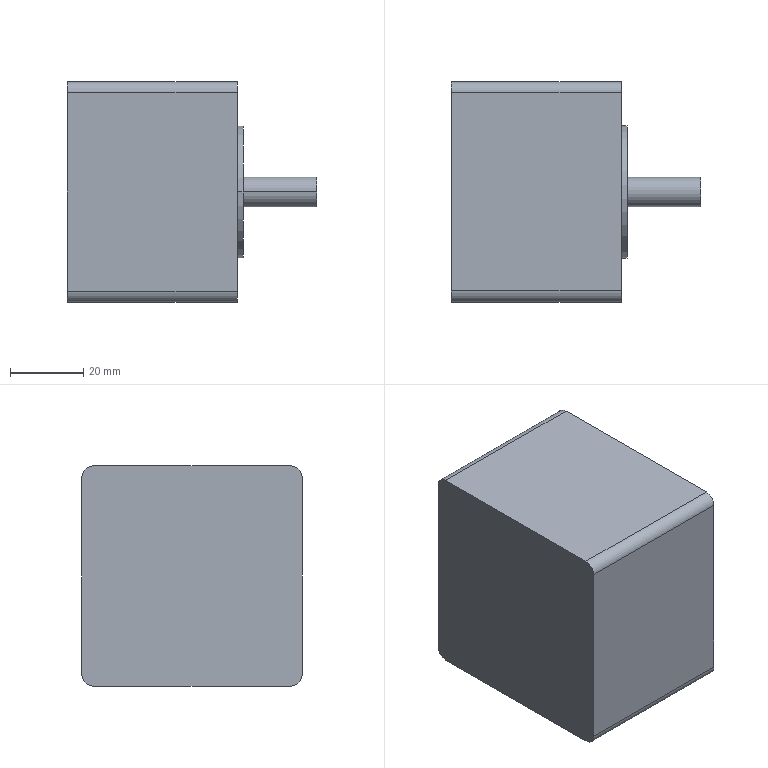Component | SolidWorks | 60Step-1 | 1 solid | 32 faces | box 67.9 x 60 x 60 mm | volume 168599 mm3 | cylinder 16 | cone 8 | plane 8 | commonest cylinder face diameters 3.3 x8 6 x4 8 x2 36 x2
build123d program:
from build123d import *

# Parameters (mm, degrees)
SKETCH1_W             = 60
SKETCH1_H             = 60
BOSS_EXTRUDE1_DEPTH   = 46.3
SKETCH2_R             = 18
BOSS_EXTRUDE2_DEPTH   = 1.6
M4_TAPPED_HOLE1_D     = 3.3
M4_TAPPED_HOLE1_DEPTH = 10.1
M4_TAPPED_HOLE1_TIP   = 0.9914
SKETCH6_R             = 4
BOSS_EXTRUDE3_DEPTH   = 20
FILLET1_R             = 3


with BuildPart() as part:
    # Sketch1 → Boss-Extrude1 (new body)
    with BuildSketch(Plane.XY):
        Rectangle(SKETCH1_W, SKETCH1_H)
    extrude(amount=BOSS_EXTRUDE1_DEPTH)

    # Sketch2 → Boss-Extrude2 (add)
    with BuildSketch(Plane.XY.offset(46.3)):
        Circle(SKETCH2_R)
    extrude(amount=BOSS_EXTRUDE2_DEPTH)

    # M4 Tapped Hole1
    with Locations(Plane.XY.offset(46.3)):
        with Locations((-25, 25), (25, 25), (25, -25), (-25, -25)):
            Hole(M4_TAPPED_HOLE1_D / 2, depth=M4_TAPPED_HOLE1_DEPTH)
            with Locations((0, 0, -(M4_TAPPED_HOLE1_DEPTH + M4_TAPPED_HOLE1_TIP / 2))):  # 118° drill point
                Cone(0, M4_TAPPED_HOLE1_D / 2, M4_TAPPED_HOLE1_TIP, mode=Mode.SUBTRACT)

    # Sketch6 → Boss-Extrude3 (add)
    with BuildSketch(Plane.XY.offset(47.9)):
        Circle(SKETCH6_R)
    extrude(amount=BOSS_EXTRUDE3_DEPTH)

    # Fillet1
    fillet1_edges = [part.edges().sort_by_distance(p)[0] for p in [
        (30, -30, 23.15),
        (-30, -30, 23.15),
        (-30, 30, 23.15),
        (30, 30, 23.15),
    ]]
    fillet(fillet1_edges, radius=FILLET1_R)


solid = part.part

# Placed as in the assembly
solid = solid.moved(Location((-74.3, -95.999, -200), (0, 90, 0)))
STEP:
#1=COLOUR_RGB('',0.7922,0.8196,0.9333);
#2=FILL_AREA_STYLE_COLOUR('',#1);
#3=FILL_AREA_STYLE('',(#2));
#4=SURFACE_STYLE_FILL_AREA(#3);
#5=SURFACE_SIDE_STYLE('',(#4));
#6=SURFACE_STYLE_USAGE(.BOTH.,#5);
#7=PRESENTATION_STYLE_ASSIGNMENT((#6));
#8=CARTESIAN_POINT('',(-0.252,-3.937,-7.874));
#9=VERTEX_POINT('',#8);
#10=CARTESIAN_POINT('',(-0.252,-3.622,-7.874));
#11=VERTEX_POINT('',#10);
#12=CARTESIAN_POINT('',(-0.252,-3.779,-7.874));
#13=DIRECTION('',(1.,0.,0.));
#14=DIRECTION('',(0.,-1.,0.));
#15=AXIS2_PLACEMENT_3D('',#12,#13,#14);
#16=CIRCLE('',#15,0.1575);
#17=EDGE_CURVE('',#9,#11,#16,.T.);
#18=ORIENTED_EDGE('',*,*,#17,.F.);
#19=CARTESIAN_POINT('',(-1.039,-3.937,-7.874));
#20=VERTEX_POINT('',#19);
#21=CARTESIAN_POINT('',(-0.252,-3.937,-7.874));
#22=DIRECTION('',(-1.,0.,0.));
#23=VECTOR('',#22,39.37);
#24=LINE('',#21,#23);
#25=EDGE_CURVE('',#9,#20,#24,.T.);
#26=ORIENTED_EDGE('',*,*,#25,.T.);
#27=CARTESIAN_POINT('',(-1.039,-3.622,-7.874));
#28=VERTEX_POINT('',#27);
#29=CARTESIAN_POINT('',(-1.039,-3.779,-7.874));
#30=DIRECTION('',(1.,0.,0.));
#31=DIRECTION('',(0.,-1.,0.));
#32=AXIS2_PLACEMENT_3D('',#29,#30,#31);
#33=CIRCLE('',#32,0.1575);
#34=EDGE_CURVE('',#20,#28,#33,.T.);
#35=ORIENTED_EDGE('',*,*,#34,.T.);
#36=CARTESIAN_POINT('',(-0.252,-3.622,-7.874));
#37=DIRECTION('',(-1.,0.,0.));
#38=VECTOR('',#37,39.37);
#39=LINE('',#36,#38);
#40=EDGE_CURVE('',#11,#28,#39,.T.);
#41=ORIENTED_EDGE('',*,*,#40,.F.);
#42=EDGE_LOOP('',(#18,#26,#35,#41));
#43=FACE_OUTER_BOUND('',#42,.T.);
#44=CARTESIAN_POINT('',(-0.252,-3.779,-7.874));
#45=DIRECTION('',(-1.,0.,0.));
#46=DIRECTION('',(0.,1.,0.));
#47=AXIS2_PLACEMENT_3D('',#44,#45,#46);
#48=CYLINDRICAL_SURFACE('',#47,0.1575);
#49=ADVANCED_FACE('',(#43),#48,.T.);
#50=CARTESIAN_POINT('',(-1.5,-2.73,-8.858));
#51=VERTEX_POINT('',#50);
#52=CARTESIAN_POINT('',(-1.5,-2.86,-8.858));
#53=VERTEX_POINT('',#52);
#54=CARTESIAN_POINT('',(-1.5,-2.795,-8.858));
#55=DIRECTION('',(1.,0.,0.));
#56=DIRECTION('',(0.,-1.,0.));
#57=AXIS2_PLACEMENT_3D('',#54,#55,#56);
#58=CIRCLE('',#57,0.06496);
#59=EDGE_CURVE('',#51,#53,#58,.T.);
#60=ORIENTED_EDGE('',*,*,#59,.F.);
#61=CARTESIAN_POINT('',(-1.102,-2.73,-8.858));
#62=VERTEX_POINT('',#61);
#63=CARTESIAN_POINT('',(-1.102,-2.73,-8.858));
#64=DIRECTION('',(1.,0.,0.));
#65=VECTOR('',#64,39.37);
#66=LINE('',#63,#65);
#67=EDGE_CURVE('',#51,#62,#66,.T.);
#68=ORIENTED_EDGE('',*,*,#67,.T.);
#69=CARTESIAN_POINT('',(-1.102,-2.86,-8.858));
#70=VERTEX_POINT('',#69);
#71=CARTESIAN_POINT('',(-1.102,-2.795,-8.858));
#72=DIRECTION('',(1.,0.,0.));
#73=DIRECTION('',(0.,-1.,0.));
#74=AXIS2_PLACEMENT_3D('',#71,#72,#73);
#75=CIRCLE('',#74,0.06496);
#76=EDGE_CURVE('',#62,#70,#75,.T.);
#77=ORIENTED_EDGE('',*,*,#76,.T.);
#78=CARTESIAN_POINT('',(-1.102,-2.86,-8.858));
#79=DIRECTION('',(1.,0.,0.));
#80=VECTOR('',#79,39.37);
#81=LINE('',#78,#80);
#82=EDGE_CURVE('',#53,#70,#81,.T.);
#83=ORIENTED_EDGE('',*,*,#82,.F.);
#84=EDGE_LOOP('',(#60,#68,#77,#83));
#85=FACE_OUTER_BOUND('',#84,.T.);
#86=CARTESIAN_POINT('',(-1.102,-2.795,-8.858));
#87=DIRECTION('',(1.,0.,0.));
#88=DIRECTION('',(0.,-1.,0.));
#89=AXIS2_PLACEMENT_3D('',#86,#87,#88);
#90=CYLINDRICAL_SURFACE('',#89,0.06496);
#91=ADVANCED_FACE('',(#85),#90,.F.);
#92=CARTESIAN_POINT('',(-1.539,-2.795,-8.858));
#93=VERTEX_POINT('',#92);
#94=CARTESIAN_POINT('',(-1.5,-2.86,-8.858));
#95=DIRECTION('',(0.515,-0.8572,-0.));
#96=VECTOR('',#95,39.37);
#97=LINE('',#94,#96);
#98=EDGE_CURVE('',#93,#53,#97,.T.);
#99=ORIENTED_EDGE('',*,*,#98,.F.);
#100=CARTESIAN_POINT('',(-1.5,-2.73,-8.858));
#101=DIRECTION('',(0.515,0.8572,0.));
#102=VECTOR('',#101,39.37);
#103=LINE('',#100,#102);
#104=EDGE_CURVE('',#93,#51,#103,.T.);
#105=ORIENTED_EDGE('',*,*,#104,.T.);
#106=ORIENTED_EDGE('',*,*,#59,.T.);
#107=EDGE_LOOP('',(#99,#105,#106));
#108=FACE_OUTER_BOUND('',#107,.T.);
#109=CARTESIAN_POINT('',(-1.5,-2.795,-8.858));
#110=DIRECTION('',(1.,0.,0.));
#111=DIRECTION('',(0.,-1.,0.));
#112=AXIS2_PLACEMENT_3D('',#109,#110,#111);
#113=CONICAL_SURFACE('',#112,0.06496,1.03);
#114=ADVANCED_FACE('',(#108),#113,.F.);
#115=CARTESIAN_POINT('',(-1.5,-4.699,-8.858));
#116=VERTEX_POINT('',#115);
#117=CARTESIAN_POINT('',(-1.5,-4.829,-8.858));
#118=VERTEX_POINT('',#117);
#119=CARTESIAN_POINT('',(-1.5,-4.764,-8.858));
#120=DIRECTION('',(1.,0.,0.));
#121=DIRECTION('',(0.,-1.,0.));
#122=AXIS2_PLACEMENT_3D('',#119,#120,#121);
#123=CIRCLE('',#122,0.06496);
#124=EDGE_CURVE('',#116,#118,#123,.T.);
#125=ORIENTED_EDGE('',*,*,#124,.F.);
#126=CARTESIAN_POINT('',(-1.102,-4.699,-8.858));
#127=VERTEX_POINT('',#126);
#128=CARTESIAN_POINT('',(-1.102,-4.699,-8.858));
#129=DIRECTION('',(1.,0.,0.));
#130=VECTOR('',#129,39.37);
#131=LINE('',#128,#130);
#132=EDGE_CURVE('',#116,#127,#131,.T.);
#133=ORIENTED_EDGE('',*,*,#132,.T.);
#134=CARTESIAN_POINT('',(-1.102,-4.829,-8.858));
#135=VERTEX_POINT('',#134);
#136=CARTESIAN_POINT('',(-1.102,-4.764,-8.858));
#137=DIRECTION('',(1.,0.,0.));
#138=DIRECTION('',(0.,-1.,0.));
#139=AXIS2_PLACEMENT_3D('',#136,#137,#138);
#140=CIRCLE('',#139,0.06496);
#141=EDGE_CURVE('',#127,#135,#140,.T.);
#142=ORIENTED_EDGE('',*,*,#141,.T.);
#143=CARTESIAN_POINT('',(-1.102,-4.829,-8.858));
#144=DIRECTION('',(1.,0.,0.));
#145=VECTOR('',#144,39.37);
#146=LINE('',#143,#145);
#147=EDGE_CURVE('',#118,#135,#146,.T.);
#148=ORIENTED_EDGE('',*,*,#147,.F.);
#149=EDGE_LOOP('',(#125,#133,#142,#148));
#150=FACE_OUTER_BOUND('',#149,.T.);
#151=CARTESIAN_POINT('',(-1.102,-4.764,-8.858));
#152=DIRECTION('',(1.,0.,0.));
#153=DIRECTION('',(0.,-1.,0.));
#154=AXIS2_PLACEMENT_3D('',#151,#152,#153);
#155=CYLINDRICAL_SURFACE('',#154,0.06496);
#156=ADVANCED_FACE('',(#150),#155,.F.);
#157=CARTESIAN_POINT('',(-1.539,-4.764,-8.858));
#158=VERTEX_POINT('',#157);
#159=CARTESIAN_POINT('',(-1.5,-4.829,-8.858));
#160=DIRECTION('',(0.515,-0.8572,-0.));
#161=VECTOR('',#160,39.37);
#162=LINE('',#159,#161);
#163=EDGE_CURVE('',#158,#118,#162,.T.);
#164=ORIENTED_EDGE('',*,*,#163,.F.);
#165=CARTESIAN_POINT('',(-1.5,-4.699,-8.858));
#166=DIRECTION('',(0.515,0.8572,0.));
#167=VECTOR('',#166,39.37);
#168=LINE('',#165,#167);
#169=EDGE_CURVE('',#158,#116,#168,.T.);
#170=ORIENTED_EDGE('',*,*,#169,.T.);
#171=ORIENTED_EDGE('',*,*,#124,.T.);
#172=EDGE_LOOP('',(#164,#170,#171));
#173=FACE_OUTER_BOUND('',#172,.T.);
#174=CARTESIAN_POINT('',(-1.5,-4.764,-8.858));
#175=DIRECTION('',(1.,0.,0.));
#176=DIRECTION('',(0.,-1.,0.));
#177=AXIS2_PLACEMENT_3D('',#174,#175,#176);
#178=CONICAL_SURFACE('',#177,0.06496,1.03);
#179=ADVANCED_FACE('',(#173),#178,.F.);
#180=CARTESIAN_POINT('',(-1.5,-4.699,-6.89));
#181=VERTEX_POINT('',#180);
#182=CARTESIAN_POINT('',(-1.5,-4.829,-6.89));
#183=VERTEX_POINT('',#182);
#184=CARTESIAN_POINT('',(-1.5,-4.764,-6.89));
#185=DIRECTION('',(1.,0.,0.));
#186=DIRECTION('',(0.,-1.,0.));
#187=AXIS2_PLACEMENT_3D('',#184,#185,#186);
#188=CIRCLE('',#187,0.06496);
#189=EDGE_CURVE('',#181,#183,#188,.T.);
#190=ORIENTED_EDGE('',*,*,#189,.F.);
#191=CARTESIAN_POINT('',(-1.102,-4.699,-6.89));
#192=VERTEX_POINT('',#191);
#193=CARTESIAN_POINT('',(-1.102,-4.699,-6.89));
#194=DIRECTION('',(1.,0.,0.));
#195=VECTOR('',#194,39.37);
#196=LINE('',#193,#195);
#197=EDGE_CURVE('',#181,#192,#196,.T.);
#198=ORIENTED_EDGE('',*,*,#197,.T.);
#199=CARTESIAN_POINT('',(-1.102,-4.829,-6.89));
#200=VERTEX_POINT('',#199);
#201=CARTESIAN_POINT('',(-1.102,-4.764,-6.89));
#202=DIRECTION('',(1.,0.,0.));
#203=DIRECTION('',(0.,-1.,0.));
#204=AXIS2_PLACEMENT_3D('',#201,#202,#203);
#205=CIRCLE('',#204,0.06496);
#206=EDGE_CURVE('',#192,#200,#205,.T.);
#207=ORIENTED_EDGE('',*,*,#206,.T.);
#208=CARTESIAN_POINT('',(-1.102,-4.829,-6.89));
#209=DIRECTION('',(1.,0.,0.));
#210=VECTOR('',#209,39.37);
#211=LINE('',#208,#210);
#212=EDGE_CURVE('',#183,#200,#211,.T.);
#213=ORIENTED_EDGE('',*,*,#212,.F.);
#214=EDGE_LOOP('',(#190,#198,#207,#213));
#215=FACE_OUTER_BOUND('',#214,.T.);
#216=CARTESIAN_POINT('',(-1.102,-4.764,-6.89));
#217=DIRECTION('',(1.,0.,0.));
#218=DIRECTION('',(0.,-1.,0.));
#219=AXIS2_PLACEMENT_3D('',#216,#217,#218);
#220=CYLINDRICAL_SURFACE('',#219,0.06496);
#221=ADVANCED_FACE('',(#215),#220,.F.);
#222=CARTESIAN_POINT('',(-1.539,-4.764,-6.89));
#223=VERTEX_POINT('',#222);
#224=CARTESIAN_POINT('',(-1.5,-4.829,-6.89));
#225=DIRECTION('',(0.515,-0.8572,-0.));
#226=VECTOR('',#225,39.37);
#227=LINE('',#224,#226);
#228=EDGE_CURVE('',#223,#183,#227,.T.);
#229=ORIENTED_EDGE('',*,*,#228,.F.);
#230=CARTESIAN_POINT('',(-1.5,-4.699,-6.89));
#231=DIRECTION('',(0.515,0.8572,0.));
#232=VECTOR('',#231,39.37);
#233=LINE('',#230,#232);
#234=EDGE_CURVE('',#223,#181,#233,.T.);
#235=ORIENTED_EDGE('',*,*,#234,.T.);
#236=ORIENTED_EDGE('',*,*,#189,.T.);
#237=EDGE_LOOP('',(#229,#235,#236));
#238=FACE_OUTER_BOUND('',#237,.T.);
#239=CARTESIAN_POINT('',(-1.5,-4.764,-6.89));
#240=DIRECTION('',(1.,0.,0.));
#241=DIRECTION('',(0.,-1.,0.));
#242=AXIS2_PLACEMENT_3D('',#239,#240,#241);
#243=CONICAL_SURFACE('',#242,0.06496,1.03);
#244=ADVANCED_FACE('',(#238),#243,.F.);
#245=CARTESIAN_POINT('',(-1.5,-2.73,-6.89));
#246=VERTEX_POINT('',#245);
#247=CARTESIAN_POINT('',(-1.5,-2.86,-6.89));
#248=VERTEX_POINT('',#247);
#249=CARTESIAN_POINT('',(-1.5,-2.795,-6.89));
#250=DIRECTION('',(1.,0.,0.));
#251=DIRECTION('',(0.,-1.,0.));
#252=AXIS2_PLACEMENT_3D('',#249,#250,#251);
#253=CIRCLE('',#252,0.06496);
#254=EDGE_CURVE('',#246,#248,#253,.T.);
#255=ORIENTED_EDGE('',*,*,#254,.F.);
#256=CARTESIAN_POINT('',(-1.102,-2.73,-6.89));
#257=VERTEX_POINT('',#256);
#258=CARTESIAN_POINT('',(-1.102,-2.73,-6.89));
#259=DIRECTION('',(1.,0.,0.));
#260=VECTOR('',#259,39.37);
#261=LINE('',#258,#260);
#262=EDGE_CURVE('',#246,#257,#261,.T.);
#263=ORIENTED_EDGE('',*,*,#262,.T.);
#264=CARTESIAN_POINT('',(-1.102,-2.86,-6.89));
#265=VERTEX_POINT('',#264);
#266=CARTESIAN_POINT('',(-1.102,-2.795,-6.89));
#267=DIRECTION('',(1.,0.,0.));
#268=DIRECTION('',(0.,-1.,0.));
#269=AXIS2_PLACEMENT_3D('',#266,#267,#268);
#270=CIRCLE('',#269,0.06496);
#271=EDGE_CURVE('',#257,#265,#270,.T.);
#272=ORIENTED_EDGE('',*,*,#271,.T.);
#273=CARTESIAN_POINT('',(-1.102,-2.86,-6.89));
#274=DIRECTION('',(1.,0.,0.));
#275=VECTOR('',#274,39.37);
#276=LINE('',#273,#275);
#277=EDGE_CURVE('',#248,#265,#276,.T.);
#278=ORIENTED_EDGE('',*,*,#277,.F.);
#279=EDGE_LOOP('',(#255,#263,#272,#278));
#280=FACE_OUTER_BOUND('',#279,.T.);
#281=CARTESIAN_POINT('',(-1.102,-2.795,-6.89));
#282=DIRECTION('',(1.,0.,0.));
#283=DIRECTION('',(0.,-1.,0.));
#284=AXIS2_PLACEMENT_3D('',#281,#282,#283);
#285=CYLINDRICAL_SURFACE('',#284,0.06496);
#286=ADVANCED_FACE('',(#280),#285,.F.);
#287=CARTESIAN_POINT('',(-1.539,-2.795,-6.89));
#288=VERTEX_POINT('',#287);
#289=CARTESIAN_POINT('',(-1.5,-2.86,-6.89));
#290=DIRECTION('',(0.515,-0.8572,-0.));
#291=VECTOR('',#290,39.37);
#292=LINE('',#289,#291);
#293=EDGE_CURVE('',#288,#248,#292,.T.);
#294=ORIENTED_EDGE('',*,*,#293,.F.);
#295=CARTESIAN_POINT('',(-1.5,-2.73,-6.89));
#296=DIRECTION('',(0.515,0.8572,0.));
#297=VECTOR('',#296,39.37);
#298=LINE('',#295,#297);
#299=EDGE_CURVE('',#288,#246,#298,.T.);
#300=ORIENTED_EDGE('',*,*,#299,.T.);
#301=ORIENTED_EDGE('',*,*,#254,.T.);
#302=EDGE_LOOP('',(#294,#300,#301));
#303=FACE_OUTER_BOUND('',#302,.T.);
#304=CARTESIAN_POINT('',(-1.5,-2.795,-6.89));
#305=DIRECTION('',(1.,0.,0.));
#306=DIRECTION('',(0.,-1.,0.));
#307=AXIS2_PLACEMENT_3D('',#304,#305,#306);
#308=CONICAL_SURFACE('',#307,0.06496,1.03);
#309=ADVANCED_FACE('',(#303),#308,.F.);
#310=CARTESIAN_POINT('',(-1.039,-4.488,-7.874));
#311=VERTEX_POINT('',#310);
#312=CARTESIAN_POINT('',(-1.039,-3.071,-7.874));
#313=VERTEX_POINT('',#312);
#314=CARTESIAN_POINT('',(-1.039,-3.779,-7.874));
#315=DIRECTION('',(1.,0.,0.));
#316=DIRECTION('',(0.,-1.,0.));
#317=AXIS2_PLACEMENT_3D('',#314,#315,#316);
#318=CIRCLE('',#317,0.7087);
#319=EDGE_CURVE('',#311,#313,#318,.T.);
#320=ORIENTED_EDGE('',*,*,#319,.F.);
#321=CARTESIAN_POINT('',(-1.102,-4.488,-7.874));
#322=VERTEX_POINT('',#321);
#323=CARTESIAN_POINT('',(-1.039,-4.488,-7.874));
#324=DIRECTION('',(-1.,0.,0.));
#325=VECTOR('',#324,39.37);
#326=LINE('',#323,#325);
#327=EDGE_CURVE('',#311,#322,#326,.T.);
#328=ORIENTED_EDGE('',*,*,#327,.T.);
#329=CARTESIAN_POINT('',(-1.102,-3.071,-7.874));
#330=VERTEX_POINT('',#329);
#331=CARTESIAN_POINT('',(-1.102,-3.779,-7.874));
#332=DIRECTION('',(1.,0.,0.));
#333=DIRECTION('',(0.,-1.,0.));
#334=AXIS2_PLACEMENT_3D('',#331,#332,#333);
#335=CIRCLE('',#334,0.7087);
#336=EDGE_CURVE('',#322,#330,#335,.T.);
#337=ORIENTED_EDGE('',*,*,#336,.T.);
#338=CARTESIAN_POINT('',(-1.039,-3.071,-7.874));
#339=DIRECTION('',(-1.,0.,0.));
#340=VECTOR('',#339,39.37);
#341=LINE('',#338,#340);
#342=EDGE_CURVE('',#313,#330,#341,.T.);
#343=ORIENTED_EDGE('',*,*,#342,.F.);
#344=EDGE_LOOP('',(#320,#328,#337,#343));
#345=FACE_OUTER_BOUND('',#344,.T.);
#346=CARTESIAN_POINT('',(-1.039,-3.779,-7.874));
#347=DIRECTION('',(-1.,0.,0.));
#348=DIRECTION('',(0.,1.,0.));
#349=AXIS2_PLACEMENT_3D('',#346,#347,#348);
#350=CYLINDRICAL_SURFACE('',#349,0.7087);
#351=ADVANCED_FACE('',(#345),#350,.T.);
#352=CARTESIAN_POINT('',(-1.102,-4.961,-6.811));
#353=VERTEX_POINT('',#352);
#354=CARTESIAN_POINT('',(-1.102,-4.961,-8.937));
#355=VERTEX_POINT('',#354);
#356=CARTESIAN_POINT('',(-1.102,-4.961,-6.693));
#357=DIRECTION('',(0.,0.,-1.));
#358=VECTOR('',#357,39.37);
#359=LINE('',#356,#358);
#360=EDGE_CURVE('',#353,#355,#359,.T.);
#361=ORIENTED_EDGE('',*,*,#360,.F.);
#362=CARTESIAN_POINT('',(-2.925,-4.961,-6.811));
#363=VERTEX_POINT('',#362);
#364=CARTESIAN_POINT('',(-1.102,-4.961,-6.811));
#365=DIRECTION('',(-1.,0.,0.));
#366=VECTOR('',#365,39.37);
#367=LINE('',#364,#366);
#368=EDGE_CURVE('',#353,#363,#367,.T.);
#369=ORIENTED_EDGE('',*,*,#368,.T.);
#370=CARTESIAN_POINT('',(-2.925,-4.961,-8.937));
#371=VERTEX_POINT('',#370);
#372=CARTESIAN_POINT('',(-2.925,-4.961,-6.693));
#373=DIRECTION('',(0.,0.,-1.));
#374=VECTOR('',#373,39.37);
#375=LINE('',#372,#374);
#376=EDGE_CURVE('',#363,#371,#375,.T.);
#377=ORIENTED_EDGE('',*,*,#376,.T.);
#378=CARTESIAN_POINT('',(-1.102,-4.961,-8.937));
#379=DIRECTION('',(1.,0.,0.));
#380=VECTOR('',#379,39.37);
#381=LINE('',#378,#380);
#382=EDGE_CURVE('',#371,#355,#381,.T.);
#383=ORIENTED_EDGE('',*,*,#382,.T.);
#384=EDGE_LOOP('',(#361,#369,#377,#383));
#385=FACE_OUTER_BOUND('',#384,.T.);
#386=CARTESIAN_POINT('',(-1.102,-4.961,-6.693));
#387=DIRECTION('',(0.,1.,0.));
#388=DIRECTION('',(1.,0.,0.));
#389=AXIS2_PLACEMENT_3D('',#386,#387,#388);
#390=PLANE('',#389);
#391=ADVANCED_FACE('',(#385),#390,.F.);
#392=CARTESIAN_POINT('',(-2.925,-4.842,-9.055));
#393=VERTEX_POINT('',#392);
#394=CARTESIAN_POINT('',(-2.925,-2.717,-9.055));
#395=VERTEX_POINT('',#394);
#396=CARTESIAN_POINT('',(-2.925,-2.598,-9.055));
#397=DIRECTION('',(0.,1.,0.));
#398=VECTOR('',#397,39.37);
#399=LINE('',#396,#398);
#400=EDGE_CURVE('',#393,#395,#399,.T.);
#401=ORIENTED_EDGE('',*,*,#400,.T.);
#402=CARTESIAN_POINT('',(-1.102,-2.717,-9.055));
#403=VERTEX_POINT('',#402);
#404=CARTESIAN_POINT('',(-1.102,-2.717,-9.055));
#405=DIRECTION('',(1.,0.,0.));
#406=VECTOR('',#405,39.37);
#407=LINE('',#404,#406);
#408=EDGE_CURVE('',#395,#403,#407,.T.);
#409=ORIENTED_EDGE('',*,*,#408,.T.);
#410=CARTESIAN_POINT('',(-1.102,-4.842,-9.055));
#411=VERTEX_POINT('',#410);
#412=CARTESIAN_POINT('',(-1.102,-2.598,-9.055));
#413=DIRECTION('',(0.,1.,0.));
#414=VECTOR('',#413,39.37);
#415=LINE('',#412,#414);
#416=EDGE_CURVE('',#411,#403,#415,.T.);
#417=ORIENTED_EDGE('',*,*,#416,.F.);
#418=CARTESIAN_POINT('',(-1.102,-4.842,-9.055));
#419=DIRECTION('',(-1.,0.,0.));
#420=VECTOR('',#419,39.37);
#421=LINE('',#418,#420);
#422=EDGE_CURVE('',#411,#393,#421,.T.);
#423=ORIENTED_EDGE('',*,*,#422,.T.);
#424=EDGE_LOOP('',(#401,#409,#417,#423));
#425=FACE_OUTER_BOUND('',#424,.T.);
#426=CARTESIAN_POINT('',(-1.102,-2.598,-9.055));
#427=DIRECTION('',(0.,-0.,1.));
#428=DIRECTION('',(-1.,0.,0.));
#429=AXIS2_PLACEMENT_3D('',#426,#427,#428);
#430=PLANE('',#429);
#431=ADVANCED_FACE('',(#425),#430,.F.);
#432=CARTESIAN_POINT('',(-2.925,-2.598,-8.937));
#433=VERTEX_POINT('',#432);
#434=CARTESIAN_POINT('',(-2.925,-2.598,-6.811));
#435=VERTEX_POINT('',#434);
#436=CARTESIAN_POINT('',(-2.925,-2.598,-6.693));
#437=DIRECTION('',(0.,-0.,1.));
#438=VECTOR('',#437,39.37);
#439=LINE('',#436,#438);
#440=EDGE_CURVE('',#433,#435,#439,.T.);
#441=ORIENTED_EDGE('',*,*,#440,.T.);
#442=CARTESIAN_POINT('',(-1.102,-2.598,-6.811));
#443=VERTEX_POINT('',#442);
#444=CARTESIAN_POINT('',(-1.102,-2.598,-6.811));
#445=DIRECTION('',(1.,0.,0.));
#446=VECTOR('',#445,39.37);
#447=LINE('',#444,#446);
#448=EDGE_CURVE('',#435,#443,#447,.T.);
#449=ORIENTED_EDGE('',*,*,#448,.T.);
#450=CARTESIAN_POINT('',(-1.102,-2.598,-8.937));
#451=VERTEX_POINT('',#450);
#452=CARTESIAN_POINT('',(-1.102,-2.598,-6.693));
#453=DIRECTION('',(0.,-0.,1.));
#454=VECTOR('',#453,39.37);
#455=LINE('',#452,#454);
#456=EDGE_CURVE('',#451,#443,#455,.T.);
#457=ORIENTED_EDGE('',*,*,#456,.F.);
#458=CARTESIAN_POINT('',(-1.102,-2.598,-8.937));
#459=DIRECTION('',(-1.,0.,0.));
#460=VECTOR('',#459,39.37);
#461=LINE('',#458,#460);
#462=EDGE_CURVE('',#451,#433,#461,.T.);
#463=ORIENTED_EDGE('',*,*,#462,.T.);
#464=EDGE_LOOP('',(#441,#449,#457,#463));
#465=FACE_OUTER_BOUND('',#464,.T.);
#466=CARTESIAN_POINT('',(-1.102,-2.598,-6.693));
#467=DIRECTION('',(0.,-1.,-0.));
#468=DIRECTION('',(-1.,0.,0.));
#469=AXIS2_PLACEMENT_3D('',#466,#467,#468);
#470=PLANE('',#469);
#471=ADVANCED_FACE('',(#465),#470,.F.);
#472=CARTESIAN_POINT('',(-2.925,-2.717,-6.693));
#473=VERTEX_POINT('',#472);
#474=CARTESIAN_POINT('',(-2.925,-4.842,-6.693));
#475=VERTEX_POINT('',#474);
#476=CARTESIAN_POINT('',(-2.925,-2.598,-6.693));
#477=DIRECTION('',(0.,-1.,-0.));
#478=VECTOR('',#477,39.37);
#479=LINE('',#476,#478);
#480=EDGE_CURVE('',#473,#475,#479,.T.);
#481=ORIENTED_EDGE('',*,*,#480,.T.);
#482=CARTESIAN_POINT('',(-1.102,-4.842,-6.693));
#483=VERTEX_POINT('',#482);
#484=CARTESIAN_POINT('',(-1.102,-4.842,-6.693));
#485=DIRECTION('',(1.,0.,0.));
#486=VECTOR('',#485,39.37);
#487=LINE('',#484,#486);
#488=EDGE_CURVE('',#475,#483,#487,.T.);
#489=ORIENTED_EDGE('',*,*,#488,.T.);
#490=CARTESIAN_POINT('',(-1.102,-2.717,-6.693));
#491=VERTEX_POINT('',#490);
#492=CARTESIAN_POINT('',(-1.102,-2.598,-6.693));
#493=DIRECTION('',(0.,-1.,-0.));
#494=VECTOR('',#493,39.37);
#495=LINE('',#492,#494);
#496=EDGE_CURVE('',#491,#483,#495,.T.);
#497=ORIENTED_EDGE('',*,*,#496,.F.);
#498=CARTESIAN_POINT('',(-1.102,-2.717,-6.693));
#499=DIRECTION('',(-1.,0.,0.));
#500=VECTOR('',#499,39.37);
#501=LINE('',#498,#500);
#502=EDGE_CURVE('',#491,#473,#501,.T.);
#503=ORIENTED_EDGE('',*,*,#502,.T.);
#504=EDGE_LOOP('',(#481,#489,#497,#503));
#505=FACE_OUTER_BOUND('',#504,.T.);
#506=CARTESIAN_POINT('',(-1.102,-2.598,-6.693));
#507=DIRECTION('',(0.,0.,-1.));
#508=DIRECTION('',(1.,0.,0.));
#509=AXIS2_PLACEMENT_3D('',#506,#507,#508);
#510=PLANE('',#509);
#511=ADVANCED_FACE('',(#505),#510,.F.);
#512=CARTESIAN_POINT('',(-1.102,-2.795,-8.858));
#513=DIRECTION('',(1.,0.,0.));
#514=DIRECTION('',(0.,-1.,0.));
#515=AXIS2_PLACEMENT_3D('',#512,#513,#514);
#516=CIRCLE('',#515,0.06496);
#517=EDGE_CURVE('',#70,#62,#516,.T.);
#518=ORIENTED_EDGE('',*,*,#517,.F.);
#519=ORIENTED_EDGE('',*,*,#76,.F.);
#520=EDGE_LOOP('',(#518,#519));
#521=FACE_BOUND('',#520,.T.);
#522=CARTESIAN_POINT('',(-1.102,-4.764,-8.858));
#523=DIRECTION('',(1.,0.,0.));
#524=DIRECTION('',(0.,-1.,0.));
#525=AXIS2_PLACEMENT_3D('',#522,#523,#524);
#526=CIRCLE('',#525,0.06496);
#527=EDGE_CURVE('',#135,#127,#526,.T.);
#528=ORIENTED_EDGE('',*,*,#527,.F.);
#529=ORIENTED_EDGE('',*,*,#141,.F.);
#530=EDGE_LOOP('',(#528,#529));
#531=FACE_BOUND('',#530,.T.);
#532=CARTESIAN_POINT('',(-1.102,-4.764,-6.89));
#533=DIRECTION('',(1.,0.,0.));
#534=DIRECTION('',(0.,-1.,0.));
#535=AXIS2_PLACEMENT_3D('',#532,#533,#534);
#536=CIRCLE('',#535,0.06496);
#537=EDGE_CURVE('',#200,#192,#536,.T.);
#538=ORIENTED_EDGE('',*,*,#537,.F.);
#539=ORIENTED_EDGE('',*,*,#206,.F.);
#540=EDGE_LOOP('',(#538,#539));
#541=FACE_BOUND('',#540,.T.);
#542=CARTESIAN_POINT('',(-1.102,-2.795,-6.89));
#543=DIRECTION('',(1.,0.,0.));
#544=DIRECTION('',(0.,-1.,0.));
#545=AXIS2_PLACEMENT_3D('',#542,#543,#544);
#546=CIRCLE('',#545,0.06496);
#547=EDGE_CURVE('',#265,#257,#546,.T.);
#548=ORIENTED_EDGE('',*,*,#547,.F.);
#549=ORIENTED_EDGE('',*,*,#271,.F.);
#550=EDGE_LOOP('',(#548,#549));
#551=FACE_BOUND('',#550,.T.);
#552=CARTESIAN_POINT('',(-1.102,-3.779,-7.874));
#553=DIRECTION('',(1.,0.,0.));
#554=DIRECTION('',(0.,-1.,0.));
#555=AXIS2_PLACEMENT_3D('',#552,#553,#554);
#556=CIRCLE('',#555,0.7087);
#557=EDGE_CURVE('',#330,#322,#556,.T.);
#558=ORIENTED_EDGE('',*,*,#557,.F.);
#559=ORIENTED_EDGE('',*,*,#336,.F.);
#560=EDGE_LOOP('',(#558,#559));
#561=FACE_BOUND('',#560,.T.);
#562=ORIENTED_EDGE('',*,*,#496,.T.);
#563=CARTESIAN_POINT('',(-1.102,-4.842,-6.811));
#564=DIRECTION('',(1.,0.,0.));
#565=DIRECTION('',(0.,1.,0.));
#566=AXIS2_PLACEMENT_3D('',#563,#564,#565);
#567=CIRCLE('',#566,0.1181);
#568=EDGE_CURVE('',#483,#353,#567,.T.);
#569=ORIENTED_EDGE('',*,*,#568,.T.);
#570=ORIENTED_EDGE('',*,*,#360,.T.);
#571=CARTESIAN_POINT('',(-1.102,-4.842,-8.937));
#572=DIRECTION('',(1.,0.,0.));
#573=DIRECTION('',(0.,1.,0.));
#574=AXIS2_PLACEMENT_3D('',#571,#572,#573);
#575=CIRCLE('',#574,0.1181);
#576=EDGE_CURVE('',#355,#411,#575,.T.);
#577=ORIENTED_EDGE('',*,*,#576,.T.);
#578=ORIENTED_EDGE('',*,*,#416,.T.);
#579=CARTESIAN_POINT('',(-1.102,-2.717,-8.937));
#580=DIRECTION('',(1.,0.,0.));
#581=DIRECTION('',(0.,1.,-0.));
#582=AXIS2_PLACEMENT_3D('',#579,#580,#581);
#583=CIRCLE('',#582,0.1181);
#584=EDGE_CURVE('',#403,#451,#583,.T.);
#585=ORIENTED_EDGE('',*,*,#584,.T.);
#586=ORIENTED_EDGE('',*,*,#456,.T.);
#587=CARTESIAN_POINT('',(-1.102,-2.717,-6.811));
#588=DIRECTION('',(1.,0.,0.));
#589=DIRECTION('',(0.,1.,0.));
#590=AXIS2_PLACEMENT_3D('',#587,#588,#589);
#591=CIRCLE('',#590,0.1181);
#592=EDGE_CURVE('',#443,#491,#591,.T.);
#593=ORIENTED_EDGE('',*,*,#592,.T.);
#594=EDGE_LOOP('',(#562,#569,#570,#577,#578,#585,#586,#593));
#595=FACE_OUTER_BOUND('',#594,.T.);
#596=CARTESIAN_POINT('',(-1.102,-3.779,-7.874));
#597=DIRECTION('',(-1.,0.,0.));
#598=DIRECTION('',(0.,1.,0.));
#599=AXIS2_PLACEMENT_3D('',#596,#597,#598);
#600=PLANE('',#599);
#601=ADVANCED_FACE('',(#521,#531,#541,#551,#561,#595),#600,.F.);
#602=ORIENTED_EDGE('',*,*,#376,.F.);
#603=CARTESIAN_POINT('',(-2.925,-4.842,-6.811));
#604=DIRECTION('',(-1.,0.,0.));
#605=DIRECTION('',(0.,1.,0.));
#606=AXIS2_PLACEMENT_3D('',#603,#604,#605);
#607=CIRCLE('',#606,0.1181);
#608=EDGE_CURVE('',#363,#475,#607,.T.);
#609=ORIENTED_EDGE('',*,*,#608,.T.);
#610=ORIENTED_EDGE('',*,*,#480,.F.);
#611=CARTESIAN_POINT('',(-2.925,-2.717,-6.811));
#612=DIRECTION('',(-1.,0.,0.));
#613=DIRECTION('',(0.,1.,0.));
#614=AXIS2_PLACEMENT_3D('',#611,#612,#613);
#615=CIRCLE('',#614,0.1181);
#616=EDGE_CURVE('',#473,#435,#615,.T.);
#617=ORIENTED_EDGE('',*,*,#616,.T.);
#618=ORIENTED_EDGE('',*,*,#440,.F.);
#619=CARTESIAN_POINT('',(-2.925,-2.717,-8.937));
#620=DIRECTION('',(-1.,0.,0.));
#621=DIRECTION('',(0.,1.,0.));
#622=AXIS2_PLACEMENT_3D('',#619,#620,#621);
#623=CIRCLE('',#622,0.1181);
#624=EDGE_CURVE('',#433,#395,#623,.T.);
#625=ORIENTED_EDGE('',*,*,#624,.T.);
#626=ORIENTED_EDGE('',*,*,#400,.F.);
#627=CARTESIAN_POINT('',(-2.925,-4.842,-8.937));
#628=DIRECTION('',(-1.,0.,0.));
#629=DIRECTION('',(0.,1.,0.));
#630=AXIS2_PLACEMENT_3D('',#627,#628,#629);
#631=CIRCLE('',#630,0.1181);
#632=EDGE_CURVE('',#393,#371,#631,.T.);
#633=ORIENTED_EDGE('',*,*,#632,.T.);
#634=EDGE_LOOP('',(#602,#609,#610,#617,#618,#625,#626,#633));
#635=FACE_OUTER_BOUND('',#634,.T.);
#636=CARTESIAN_POINT('',(-2.925,-3.779,-7.874));
#637=DIRECTION('',(-1.,0.,0.));
#638=DIRECTION('',(0.,1.,0.));
#639=AXIS2_PLACEMENT_3D('',#636,#637,#638);
#640=PLANE('',#639);
#641=ADVANCED_FACE('',(#635),#640,.T.);
#642=ORIENTED_EDGE('',*,*,#327,.F.);
#643=CARTESIAN_POINT('',(-1.039,-3.779,-7.874));
#644=DIRECTION('',(1.,0.,0.));
#645=DIRECTION('',(0.,-1.,0.));
#646=AXIS2_PLACEMENT_3D('',#643,#644,#645);
#647=CIRCLE('',#646,0.7087);
#648=EDGE_CURVE('',#313,#311,#647,.T.);
#649=ORIENTED_EDGE('',*,*,#648,.F.);
#650=ORIENTED_EDGE('',*,*,#342,.T.);
#651=ORIENTED_EDGE('',*,*,#557,.T.);
#652=EDGE_LOOP('',(#642,#649,#650,#651));
#653=FACE_OUTER_BOUND('',#652,.T.);
#654=CARTESIAN_POINT('',(-1.039,-3.779,-7.874));
#655=DIRECTION('',(-1.,0.,0.));
#656=DIRECTION('',(0.,1.,0.));
#657=AXIS2_PLACEMENT_3D('',#654,#655,#656);
#658=CYLINDRICAL_SURFACE('',#657,0.7087);
#659=ADVANCED_FACE('',(#653),#658,.T.);
#660=CARTESIAN_POINT('',(-1.039,-3.779,-7.874));
#661=DIRECTION('',(1.,0.,0.));
#662=DIRECTION('',(0.,-1.,0.));
#663=AXIS2_PLACEMENT_3D('',#660,#661,#662);
#664=CIRCLE('',#663,0.1575);
#665=EDGE_CURVE('',#28,#20,#664,.T.);
#666=ORIENTED_EDGE('',*,*,#665,.F.);
#667=ORIENTED_EDGE('',*,*,#34,.F.);
#668=EDGE_LOOP('',(#666,#667));
#669=FACE_BOUND('',#668,.T.);
#670=ORIENTED_EDGE('',*,*,#648,.T.);
#671=ORIENTED_EDGE('',*,*,#319,.T.);
#672=EDGE_LOOP('',(#670,#671));
#673=FACE_OUTER_BOUND('',#672,.T.);
#674=CARTESIAN_POINT('',(-1.039,-3.779,-7.874));
#675=DIRECTION('',(1.,0.,0.));
#676=DIRECTION('',(0.,-1.,-0.));
#677=AXIS2_PLACEMENT_3D('',#674,#675,#676);
#678=PLANE('',#677);
#679=ADVANCED_FACE('',(#669,#673),#678,.T.);
#680=ORIENTED_EDGE('',*,*,#299,.F.);
#681=ORIENTED_EDGE('',*,*,#293,.T.);
#682=CARTESIAN_POINT('',(-1.5,-2.795,-6.89));
#683=DIRECTION('',(1.,0.,0.));
#684=DIRECTION('',(0.,-1.,0.));
#685=AXIS2_PLACEMENT_3D('',#682,#683,#684);
#686=CIRCLE('',#685,0.06496);
#687=EDGE_CURVE('',#248,#246,#686,.T.);
#688=ORIENTED_EDGE('',*,*,#687,.T.);
#689=EDGE_LOOP('',(#680,#681,#688));
#690=FACE_OUTER_BOUND('',#689,.T.);
#691=CARTESIAN_POINT('',(-1.5,-2.795,-6.89));
#692=DIRECTION('',(1.,0.,0.));
#693=DIRECTION('',(0.,-1.,0.));
#694=AXIS2_PLACEMENT_3D('',#691,#692,#693);
#695=CONICAL_SURFACE('',#694,0.06496,1.03);
#696=ADVANCED_FACE('',(#690),#695,.F.);
#697=ORIENTED_EDGE('',*,*,#262,.F.);
#698=ORIENTED_EDGE('',*,*,#687,.F.);
#699=ORIENTED_EDGE('',*,*,#277,.T.);
#700=ORIENTED_EDGE('',*,*,#547,.T.);
#701=EDGE_LOOP('',(#697,#698,#699,#700));
#702=FACE_OUTER_BOUND('',#701,.T.);
#703=CARTESIAN_POINT('',(-1.102,-2.795,-6.89));
#704=DIRECTION('',(1.,0.,0.));
#705=DIRECTION('',(0.,-1.,0.));
#706=AXIS2_PLACEMENT_3D('',#703,#704,#705);
#707=CYLINDRICAL_SURFACE('',#706,0.06496);
#708=ADVANCED_FACE('',(#702),#707,.F.);
#709=ORIENTED_EDGE('',*,*,#234,.F.);
#710=ORIENTED_EDGE('',*,*,#228,.T.);
#711=CARTESIAN_POINT('',(-1.5,-4.764,-6.89));
#712=DIRECTION('',(1.,0.,0.));
#713=DIRECTION('',(0.,-1.,0.));
#714=AXIS2_PLACEMENT_3D('',#711,#712,#713);
#715=CIRCLE('',#714,0.06496);
#716=EDGE_CURVE('',#183,#181,#715,.T.);
#717=ORIENTED_EDGE('',*,*,#716,.T.);
#718=EDGE_LOOP('',(#709,#710,#717));
#719=FACE_OUTER_BOUND('',#718,.T.);
#720=CARTESIAN_POINT('',(-1.5,-4.764,-6.89));
#721=DIRECTION('',(1.,0.,0.));
#722=DIRECTION('',(0.,-1.,0.));
#723=AXIS2_PLACEMENT_3D('',#720,#721,#722);
#724=CONICAL_SURFACE('',#723,0.06496,1.03);
#725=ADVANCED_FACE('',(#719),#724,.F.);
#726=ORIENTED_EDGE('',*,*,#197,.F.);
#727=ORIENTED_EDGE('',*,*,#716,.F.);
#728=ORIENTED_EDGE('',*,*,#212,.T.);
#729=ORIENTED_EDGE('',*,*,#537,.T.);
#730=EDGE_LOOP('',(#726,#727,#728,#729));
#731=FACE_OUTER_BOUND('',#730,.T.);
#732=CARTESIAN_POINT('',(-1.102,-4.764,-6.89));
#733=DIRECTION('',(1.,0.,0.));
#734=DIRECTION('',(0.,-1.,0.));
#735=AXIS2_PLACEMENT_3D('',#732,#733,#734);
#736=CYLINDRICAL_SURFACE('',#735,0.06496);
#737=ADVANCED_FACE('',(#731),#736,.F.);
#738=ORIENTED_EDGE('',*,*,#169,.F.);
#739=ORIENTED_EDGE('',*,*,#163,.T.);
#740=CARTESIAN_POINT('',(-1.5,-4.764,-8.858));
#741=DIRECTION('',(1.,0.,0.));
#742=DIRECTION('',(0.,-1.,0.));
#743=AXIS2_PLACEMENT_3D('',#740,#741,#742);
#744=CIRCLE('',#743,0.06496);
#745=EDGE_CURVE('',#118,#116,#744,.T.);
#746=ORIENTED_EDGE('',*,*,#745,.T.);
#747=EDGE_LOOP('',(#738,#739,#746));
#748=FACE_OUTER_BOUND('',#747,.T.);
#749=CARTESIAN_POINT('',(-1.5,-4.764,-8.858));
#750=DIRECTION('',(1.,0.,0.));
#751=DIRECTION('',(0.,-1.,0.));
#752=AXIS2_PLACEMENT_3D('',#749,#750,#751);
#753=CONICAL_SURFACE('',#752,0.06496,1.03);
#754=ADVANCED_FACE('',(#748),#753,.F.);
#755=ORIENTED_EDGE('',*,*,#132,.F.);
#756=ORIENTED_EDGE('',*,*,#745,.F.);
#757=ORIENTED_EDGE('',*,*,#147,.T.);
#758=ORIENTED_EDGE('',*,*,#527,.T.);
#759=EDGE_LOOP('',(#755,#756,#757,#758));
#760=FACE_OUTER_BOUND('',#759,.T.);
#761=CARTESIAN_POINT('',(-1.102,-4.764,-8.858));
#762=DIRECTION('',(1.,0.,0.));
#763=DIRECTION('',(0.,-1.,0.));
#764=AXIS2_PLACEMENT_3D('',#761,#762,#763);
#765=CYLINDRICAL_SURFACE('',#764,0.06496);
#766=ADVANCED_FACE('',(#760),#765,.F.);
#767=ORIENTED_EDGE('',*,*,#104,.F.);
#768=ORIENTED_EDGE('',*,*,#98,.T.);
#769=CARTESIAN_POINT('',(-1.5,-2.795,-8.858));
#770=DIRECTION('',(1.,0.,0.));
#771=DIRECTION('',(0.,-1.,0.));
#772=AXIS2_PLACEMENT_3D('',#769,#770,#771);
#773=CIRCLE('',#772,0.06496);
#774=EDGE_CURVE('',#53,#51,#773,.T.);
#775=ORIENTED_EDGE('',*,*,#774,.T.);
#776=EDGE_LOOP('',(#767,#768,#775));
#777=FACE_OUTER_BOUND('',#776,.T.);
#778=CARTESIAN_POINT('',(-1.5,-2.795,-8.858));
#779=DIRECTION('',(1.,0.,0.));
#780=DIRECTION('',(0.,-1.,0.));
#781=AXIS2_PLACEMENT_3D('',#778,#779,#780);
#782=CONICAL_SURFACE('',#781,0.06496,1.03);
#783=ADVANCED_FACE('',(#777),#782,.F.);
#784=ORIENTED_EDGE('',*,*,#67,.F.);
#785=ORIENTED_EDGE('',*,*,#774,.F.);
#786=ORIENTED_EDGE('',*,*,#82,.T.);
#787=ORIENTED_EDGE('',*,*,#517,.T.);
#788=EDGE_LOOP('',(#784,#785,#786,#787));
#789=FACE_OUTER_BOUND('',#788,.T.);
#790=CARTESIAN_POINT('',(-1.102,-2.795,-8.858));
#791=DIRECTION('',(1.,0.,0.));
#792=DIRECTION('',(0.,-1.,0.));
#793=AXIS2_PLACEMENT_3D('',#790,#791,#792);
#794=CYLINDRICAL_SURFACE('',#793,0.06496);
#795=ADVANCED_FACE('',(#789),#794,.F.);
#796=ORIENTED_EDGE('',*,*,#25,.F.);
#797=CARTESIAN_POINT('',(-0.252,-3.779,-7.874));
#798=DIRECTION('',(1.,0.,0.));
#799=DIRECTION('',(0.,-1.,0.));
#800=AXIS2_PLACEMENT_3D('',#797,#798,#799);
#801=CIRCLE('',#800,0.1575);
#802=EDGE_CURVE('',#11,#9,#801,.T.);
#803=ORIENTED_EDGE('',*,*,#802,.F.);
#804=ORIENTED_EDGE('',*,*,#40,.T.);
#805=ORIENTED_EDGE('',*,*,#665,.T.);
#806=EDGE_LOOP('',(#796,#803,#804,#805));
#807=FACE_OUTER_BOUND('',#806,.T.);
#808=CARTESIAN_POINT('',(-0.252,-3.779,-7.874));
#809=DIRECTION('',(-1.,0.,0.));
#810=DIRECTION('',(0.,1.,0.));
#811=AXIS2_PLACEMENT_3D('',#808,#809,#810);
#812=CYLINDRICAL_SURFACE('',#811,0.1575);
#813=ADVANCED_FACE('',(#807),#812,.T.);
#814=ORIENTED_EDGE('',*,*,#802,.T.);
#815=ORIENTED_EDGE('',*,*,#17,.T.);
#816=EDGE_LOOP('',(#814,#815));
#817=FACE_OUTER_BOUND('',#816,.T.);
#818=CARTESIAN_POINT('',(-0.252,-3.779,-7.874));
#819=DIRECTION('',(1.,0.,0.));
#820=DIRECTION('',(0.,-1.,-0.));
#821=AXIS2_PLACEMENT_3D('',#818,#819,#820);
#822=PLANE('',#821);
#823=ADVANCED_FACE('',(#817),#822,.T.);
#824=ORIENTED_EDGE('',*,*,#568,.F.);
#825=ORIENTED_EDGE('',*,*,#488,.F.);
#826=ORIENTED_EDGE('',*,*,#608,.F.);
#827=ORIENTED_EDGE('',*,*,#368,.F.);
#828=EDGE_LOOP('',(#824,#825,#826,#827));
#829=FACE_OUTER_BOUND('',#828,.T.);
#830=CARTESIAN_POINT('',(-1.102,-4.842,-6.811));
#831=DIRECTION('',(-1.,0.,0.));
#832=DIRECTION('',(0.,1.,0.));
#833=AXIS2_PLACEMENT_3D('',#830,#831,#832);
#834=CYLINDRICAL_SURFACE('',#833,0.1181);
#835=ADVANCED_FACE('',(#829),#834,.T.);
#836=ORIENTED_EDGE('',*,*,#592,.F.);
#837=ORIENTED_EDGE('',*,*,#448,.F.);
#838=ORIENTED_EDGE('',*,*,#616,.F.);
#839=ORIENTED_EDGE('',*,*,#502,.F.);
#840=EDGE_LOOP('',(#836,#837,#838,#839));
#841=FACE_OUTER_BOUND('',#840,.T.);
#842=CARTESIAN_POINT('',(-1.102,-2.717,-6.811));
#843=DIRECTION('',(-1.,0.,0.));
#844=DIRECTION('',(0.,1.,0.));
#845=AXIS2_PLACEMENT_3D('',#842,#843,#844);
#846=CYLINDRICAL_SURFACE('',#845,0.1181);
#847=ADVANCED_FACE('',(#841),#846,.T.);
#848=ORIENTED_EDGE('',*,*,#584,.F.);
#849=ORIENTED_EDGE('',*,*,#408,.F.);
#850=ORIENTED_EDGE('',*,*,#624,.F.);
#851=ORIENTED_EDGE('',*,*,#462,.F.);
#852=EDGE_LOOP('',(#848,#849,#850,#851));
#853=FACE_OUTER_BOUND('',#852,.T.);
#854=CARTESIAN_POINT('',(-1.102,-2.717,-8.937));
#855=DIRECTION('',(-1.,0.,0.));
#856=DIRECTION('',(0.,1.,0.));
#857=AXIS2_PLACEMENT_3D('',#854,#855,#856);
#858=CYLINDRICAL_SURFACE('',#857,0.1181);
#859=ADVANCED_FACE('',(#853),#858,.T.);
#860=ORIENTED_EDGE('',*,*,#576,.F.);
#861=ORIENTED_EDGE('',*,*,#382,.F.);
#862=ORIENTED_EDGE('',*,*,#632,.F.);
#863=ORIENTED_EDGE('',*,*,#422,.F.);
#864=EDGE_LOOP('',(#860,#861,#862,#863));
#865=FACE_OUTER_BOUND('',#864,.T.);
#866=CARTESIAN_POINT('',(-1.102,-4.842,-8.937));
#867=DIRECTION('',(-1.,0.,0.));
#868=DIRECTION('',(0.,1.,0.));
#869=AXIS2_PLACEMENT_3D('',#866,#867,#868);
#870=CYLINDRICAL_SURFACE('',#869,0.1181);
#871=ADVANCED_FACE('',(#865),#870,.T.);
#872=CLOSED_SHELL('',(#49,#91,#114,#156,#179,#221,#244,#286,#309,#351,#391,#431,#471,#511,#601,#641,#659,#679,#696,#708,#725,#737,#754,#766,#783,#795,#813,#823,#835,#847,#859,#871));
#873=MANIFOLD_SOLID_BREP('',#872);
#874=STYLED_ITEM('',(#7),#873);
#875=PRESENTATION_LAYER_ASSIGNMENT('','',(#874));
#876=CARTESIAN_POINT('',(0.,0.,0.));
#877=DIRECTION('',(0.,0.,1.));
#878=DIRECTION('',(1.,0.,0.));
#879=AXIS2_PLACEMENT_3D('',#876,#877,#878);
#880=(LENGTH_UNIT()NAMED_UNIT(*)SI_UNIT($,.METRE.));
#881=LENGTH_MEASURE_WITH_UNIT(LENGTH_MEASURE(0.0254),#880);
#882=DIMENSIONAL_EXPONENTS(1.,0.,0.,0.,0.,0.,0.);
#883=(CONVERSION_BASED_UNIT('',#881)LENGTH_UNIT()NAMED_UNIT(#882));
#884=UNCERTAINTY_MEASURE_WITH_UNIT(LENGTH_MEASURE(0.00001),#883,'','');
#885=(NAMED_UNIT(*)PLANE_ANGLE_UNIT()SI_UNIT($,.RADIAN.));
#886=(NAMED_UNIT(*)SI_UNIT($,.STERADIAN.)SOLID_ANGLE_UNIT());
#887=(GEOMETRIC_REPRESENTATION_CONTEXT(3)GLOBAL_UNCERTAINTY_ASSIGNED_CONTEXT((#884))GLOBAL_UNIT_ASSIGNED_CONTEXT((#883,#885,#886))REPRESENTATION_CONTEXT('',''));
#888=ADVANCED_BREP_SHAPE_REPRESENTATION('',(#873,#879),#887);
#889=(LENGTH_UNIT()NAMED_UNIT(*)SI_UNIT($,.METRE.));
#890=LENGTH_MEASURE_WITH_UNIT(LENGTH_MEASURE(0.0254),#889);
#891=DIMENSIONAL_EXPONENTS(1.,0.,0.,0.,0.,0.,0.);
#892=(CONVERSION_BASED_UNIT('',#890)LENGTH_UNIT()NAMED_UNIT(#891));
#893=UNCERTAINTY_MEASURE_WITH_UNIT(LENGTH_MEASURE(0.00001),#892,'','');
#894=(NAMED_UNIT(*)PLANE_ANGLE_UNIT()SI_UNIT($,.RADIAN.));
#895=(NAMED_UNIT(*)SI_UNIT($,.STERADIAN.)SOLID_ANGLE_UNIT());
#896=(GEOMETRIC_REPRESENTATION_CONTEXT(3)GLOBAL_UNCERTAINTY_ASSIGNED_CONTEXT((#893))GLOBAL_UNIT_ASSIGNED_CONTEXT((#892,#894,#895))REPRESENTATION_CONTEXT('',''));
#897=MECHANICAL_DESIGN_GEOMETRIC_PRESENTATION_REPRESENTATION('',(#874),#896);